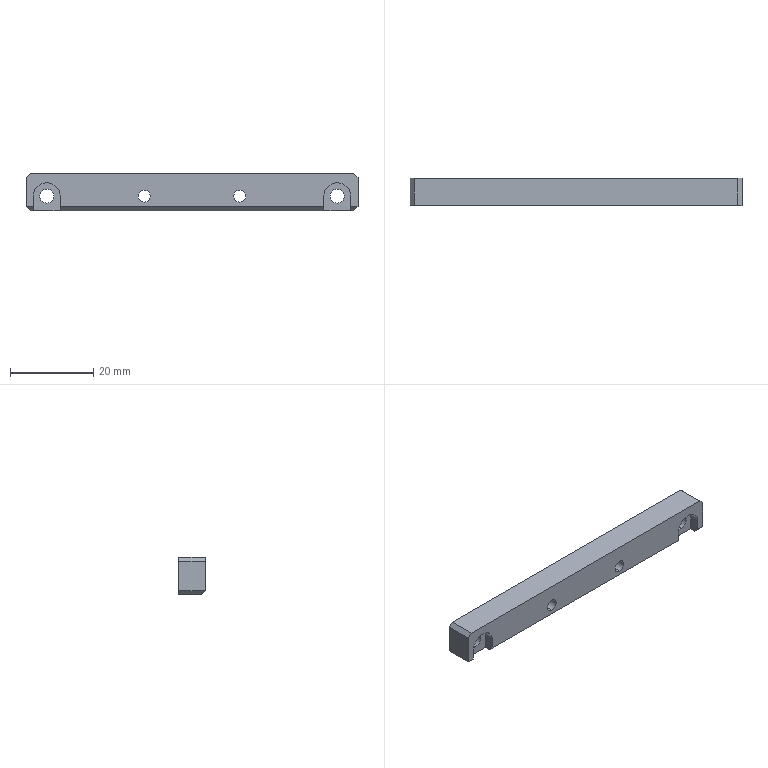CAM job | Mastercam | mm | 16 operations | part box 80 x 6.5 x 9
1. Contour (Ramp) | 6 - 6 平底刀
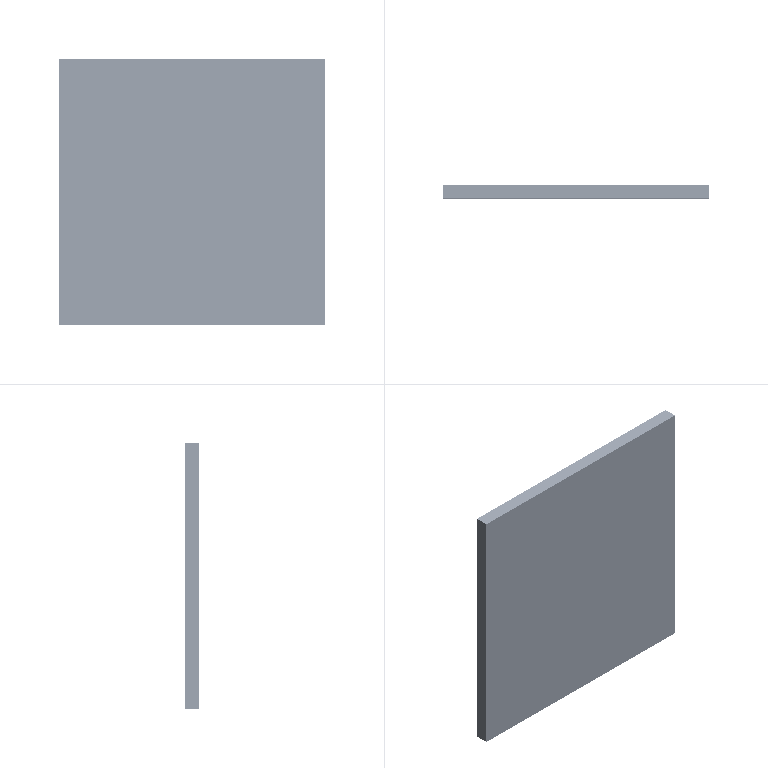2. Drill/Counterbore | 2 - 4定位倒角
3. Peck Drill | 12 - 3.4 钻头
4. Peck Drill | 13 - 2.9 钻头
5. Helix Bore | 7 - 4 平底刀
6. Facing | 8 - 6 J平底刀
7. Model Chamfer | 2 - 4定位倒角
8. Contour (Ramp) | 6 - 6 平底刀
9. Contour (2D) | 8 - 6 J平底刀
10. Facing | 9 - 10C 平底刀
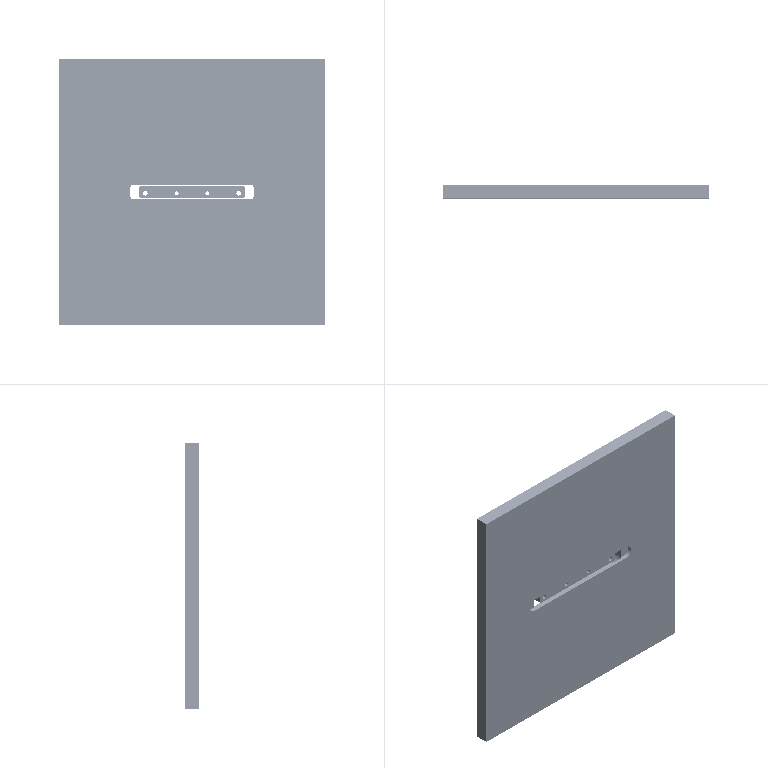11. Contour (Ramp) | 7 - 4 平底刀
12. Facing | 10 - 10J 平底刀
13. Contour (2D) | 7 - 4 平底刀
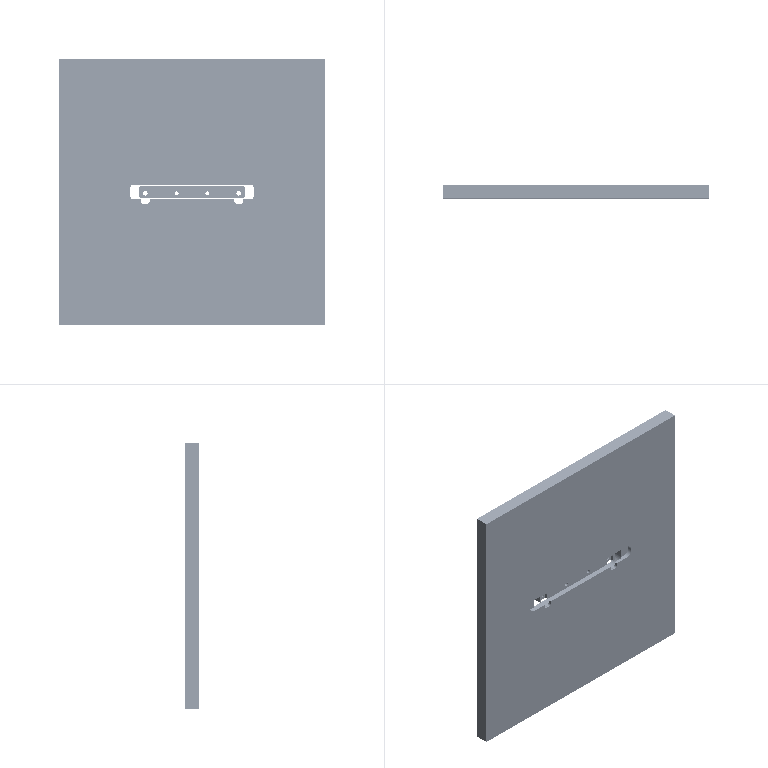14. Model Chamfer | 2 - 4定位倒角
15. Contour (2D chamfer) | 2 - 4定位倒角
16. Facing | 10 - 10J 平底刀